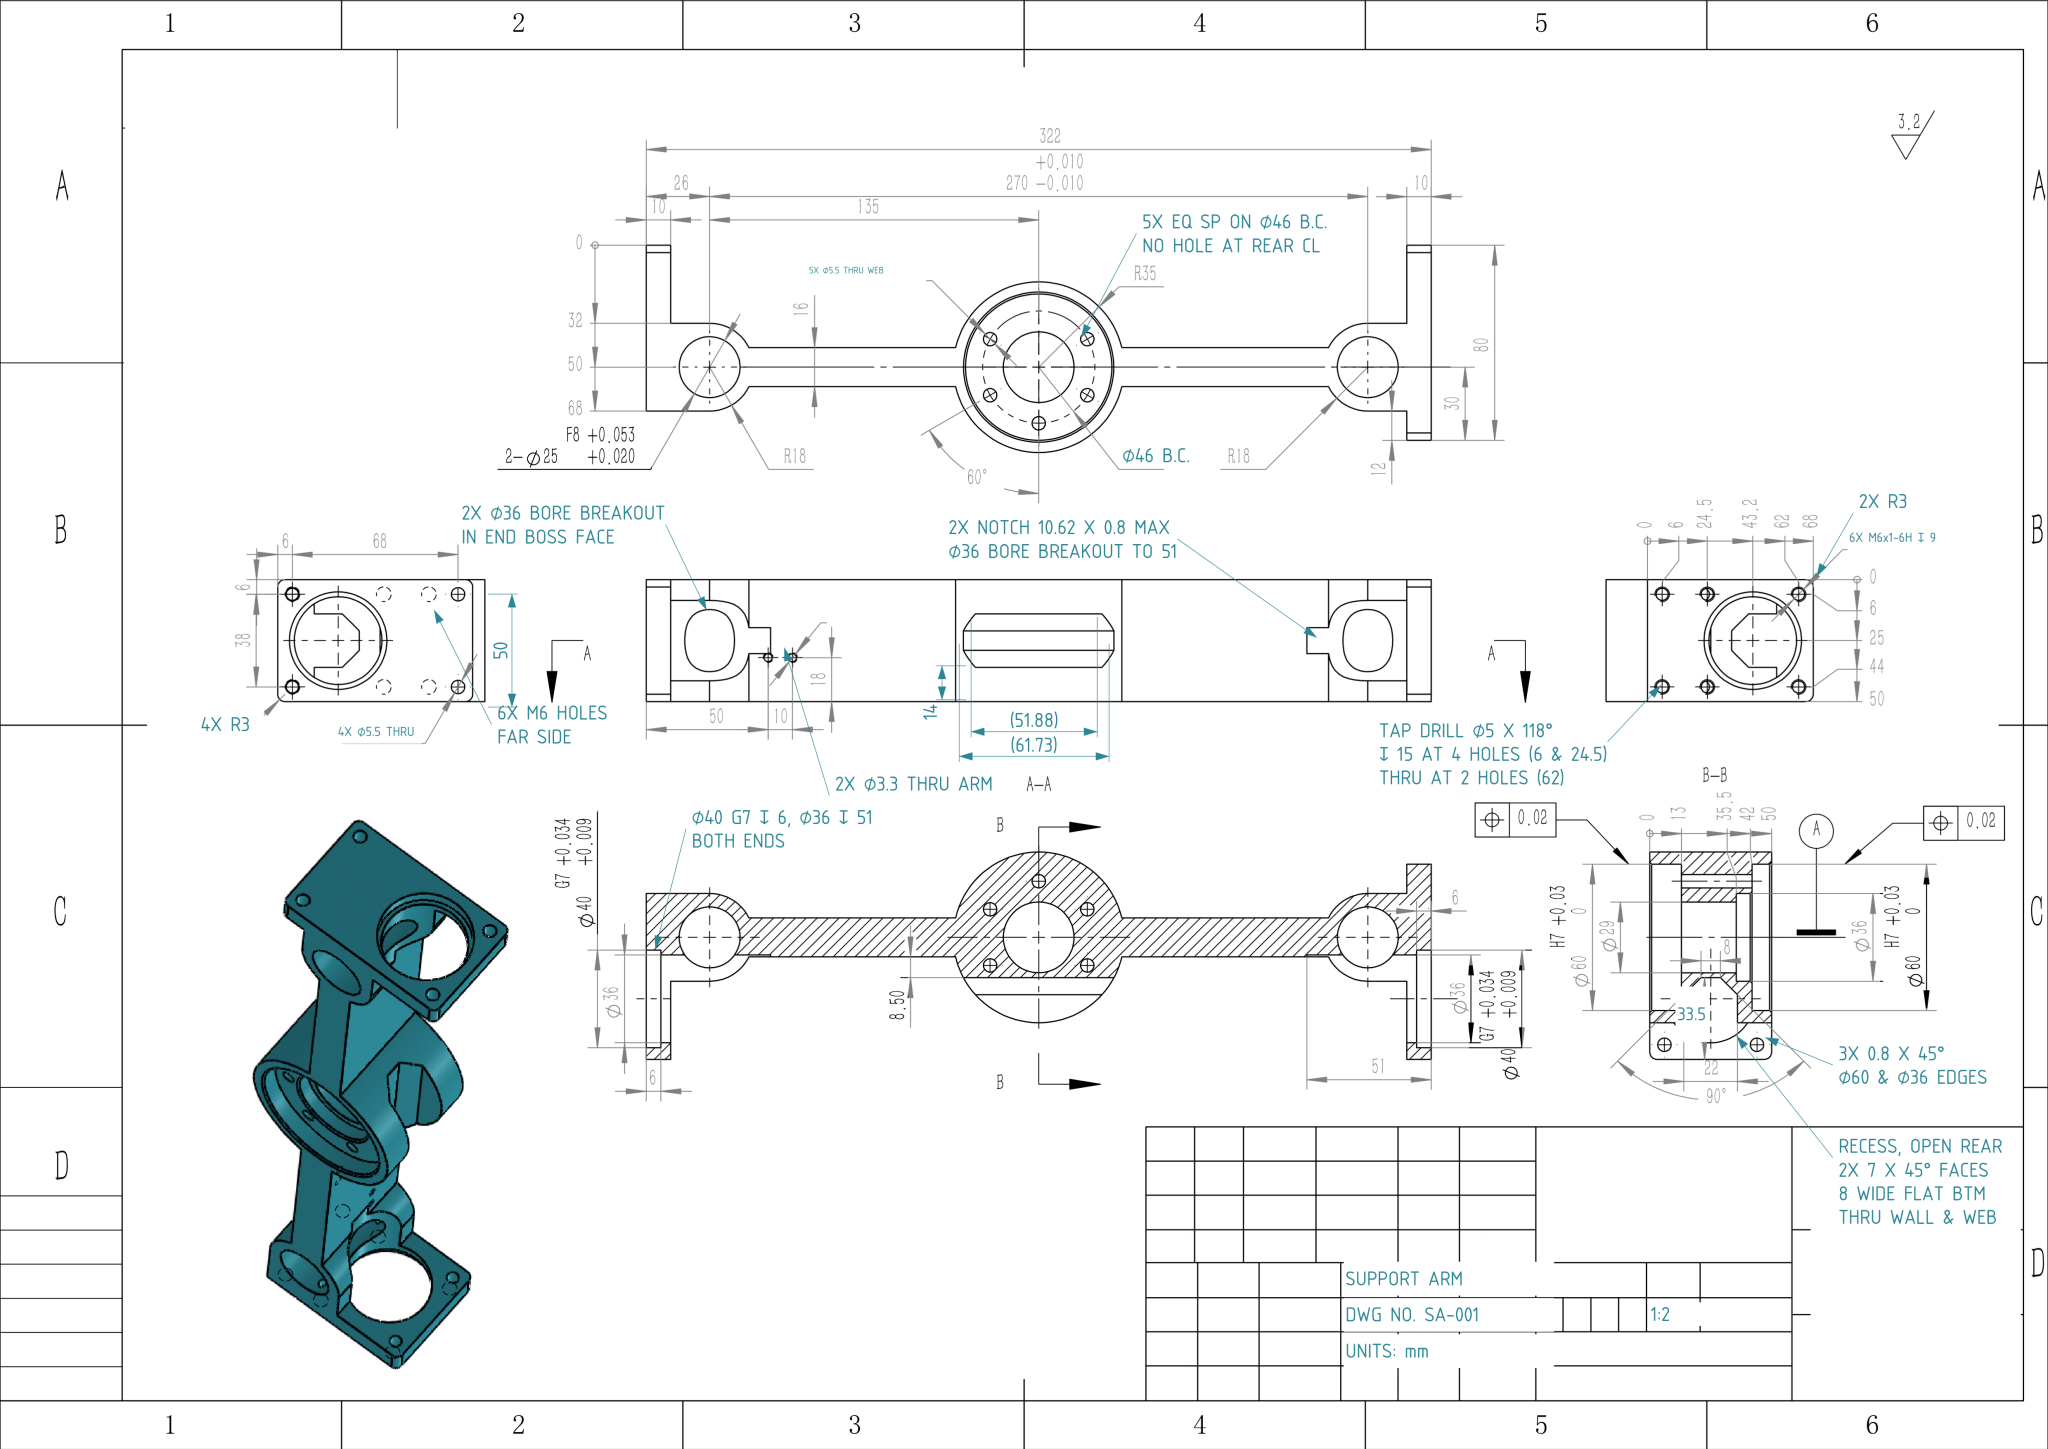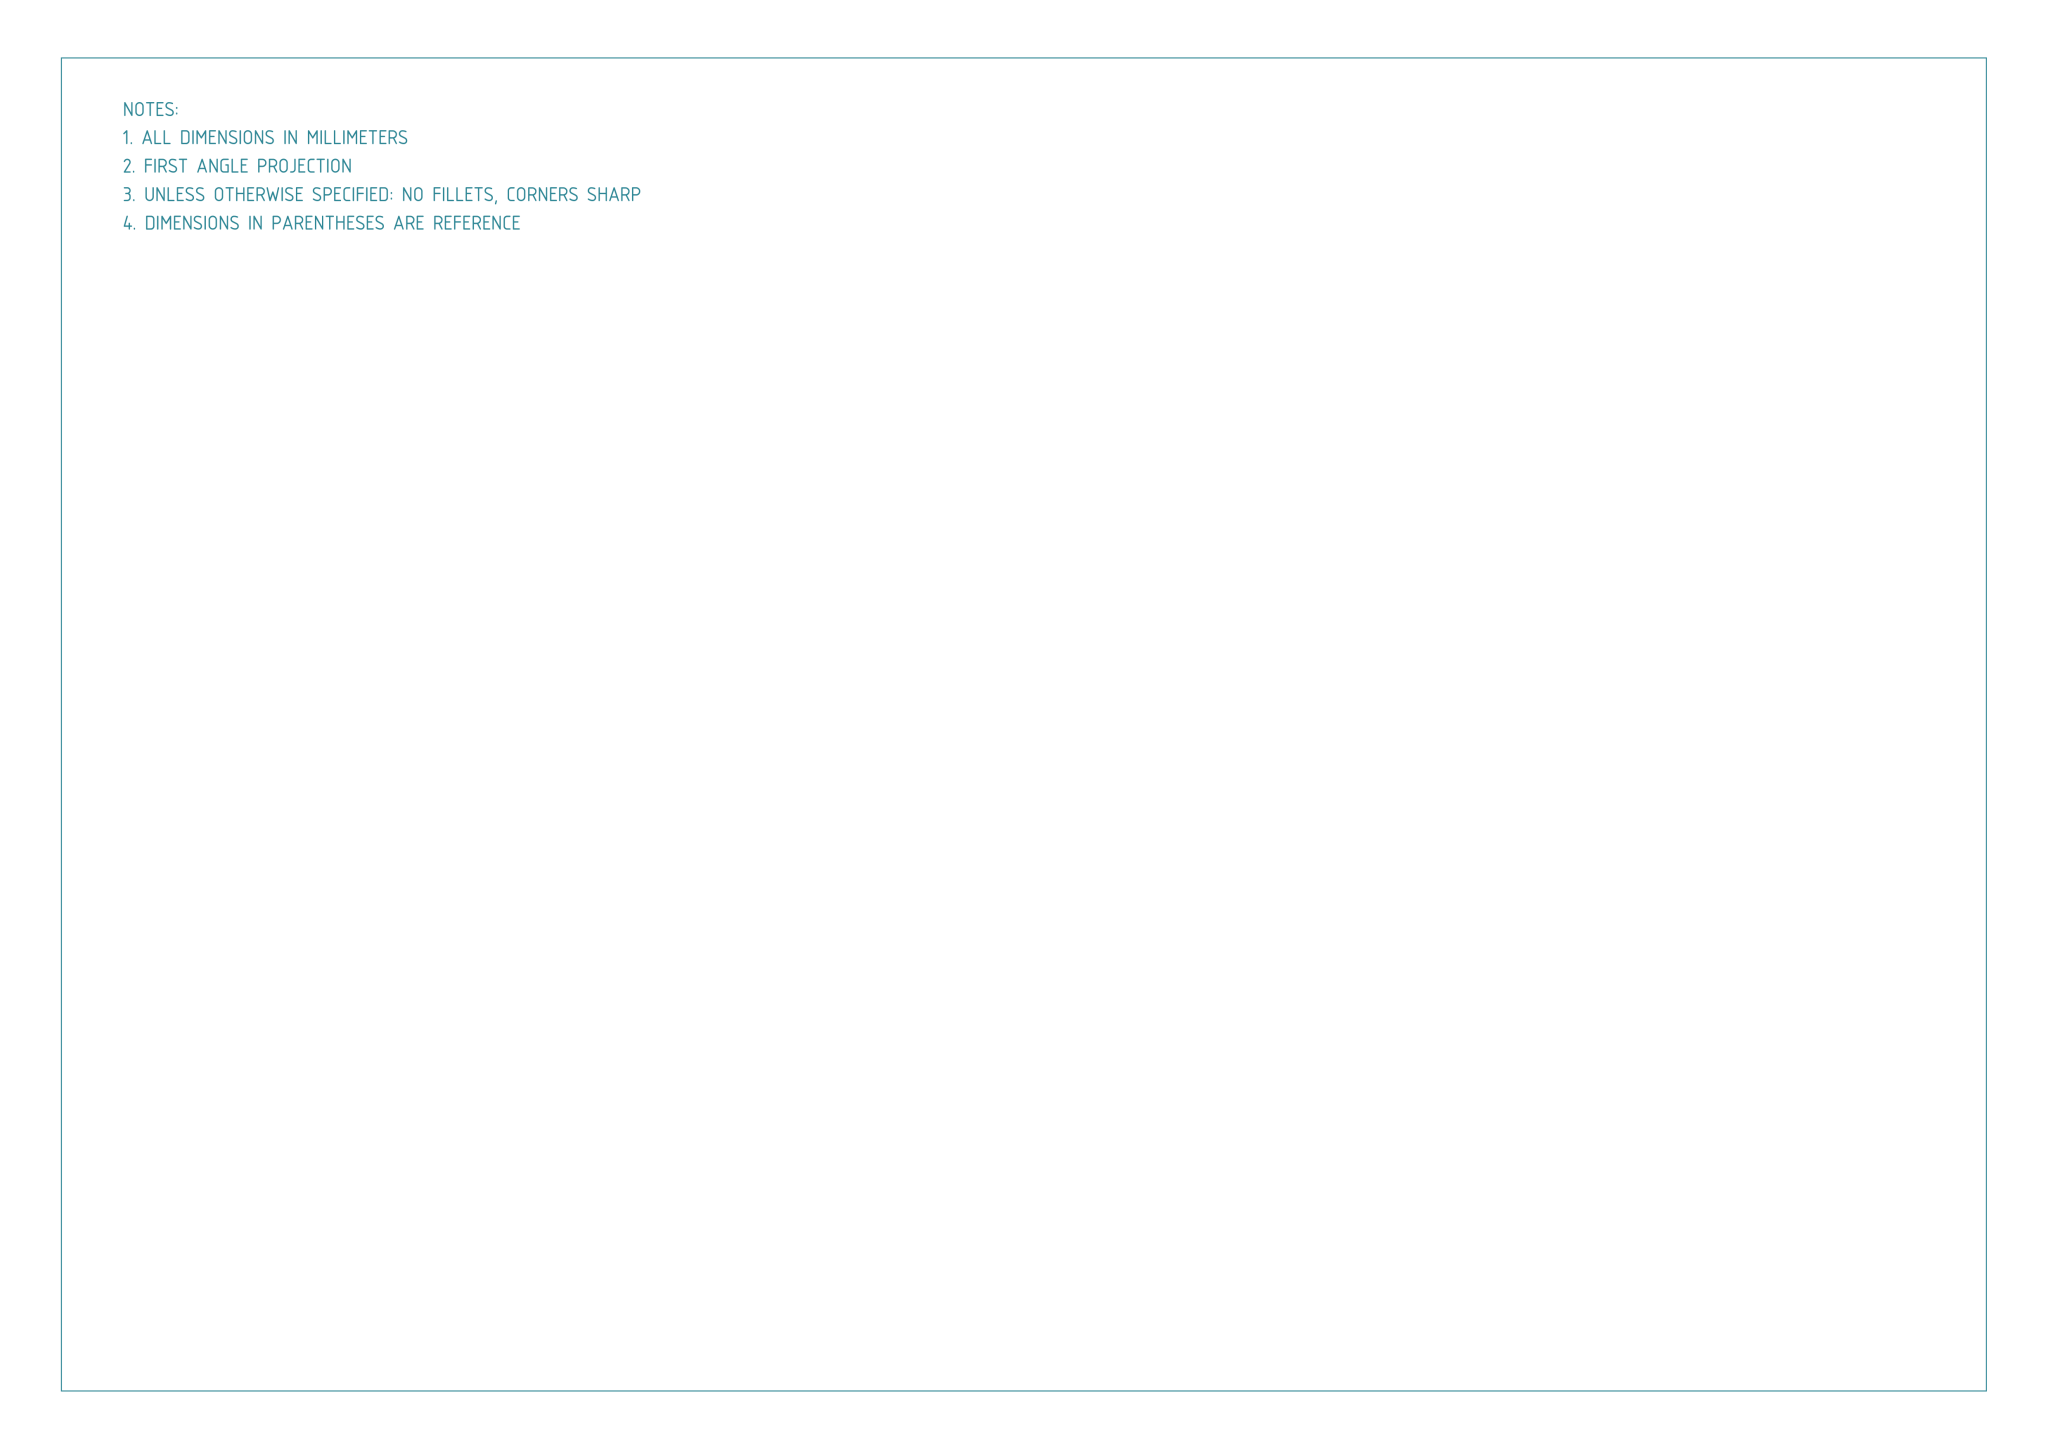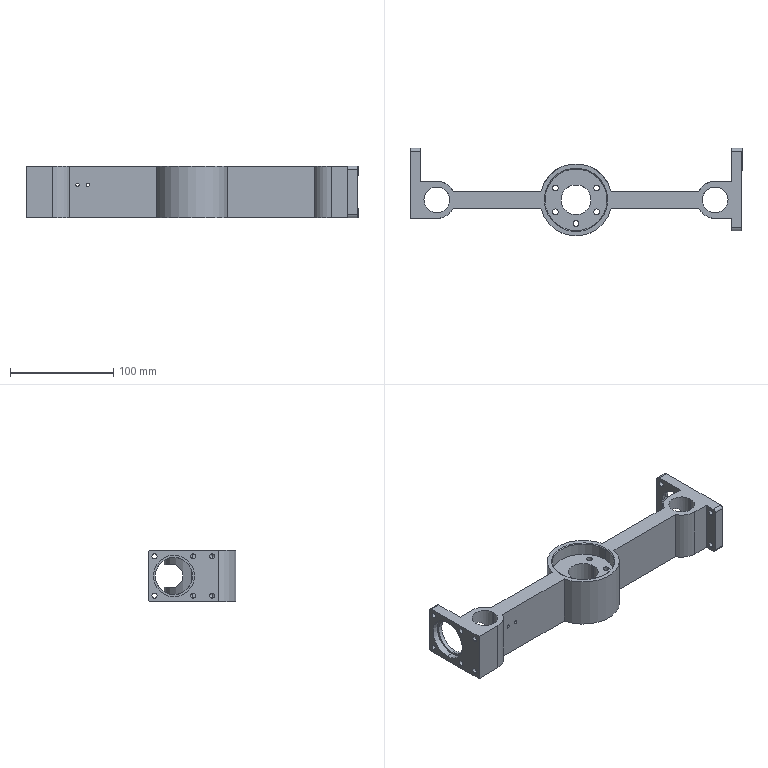Part | NX | mm | 1 solid | 116 faces | box 322 x 85 x 50 mm | volume 321372 mm3 | cylinder 68 | plane 32 | cone 16 | commonest cylinder face diameters 5.5 x18 5 x12 36 x9 6 x6 60 x4 3.3 x4 40 x4 25 x4